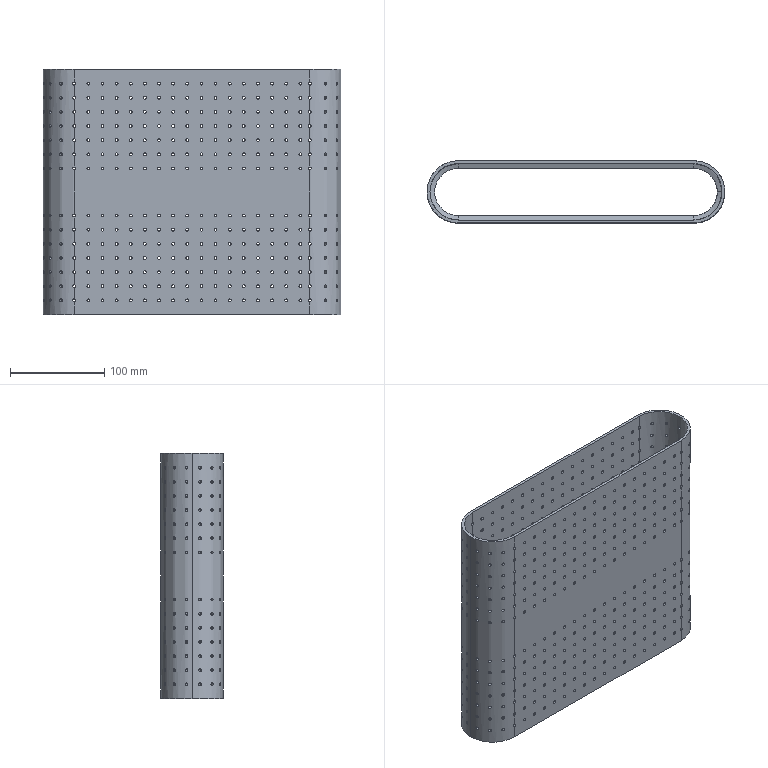Component | SolidWorks | LD101-02--Q1017-Q1-2-1 | 1 solid | 1390 faces | volume 550650 mm3 | cylinder 1356 | plane 28 | cone 6 | commonest cylinder face diameters 3 x1344 60 x6 50 x3 66 x3 | material POM (White)